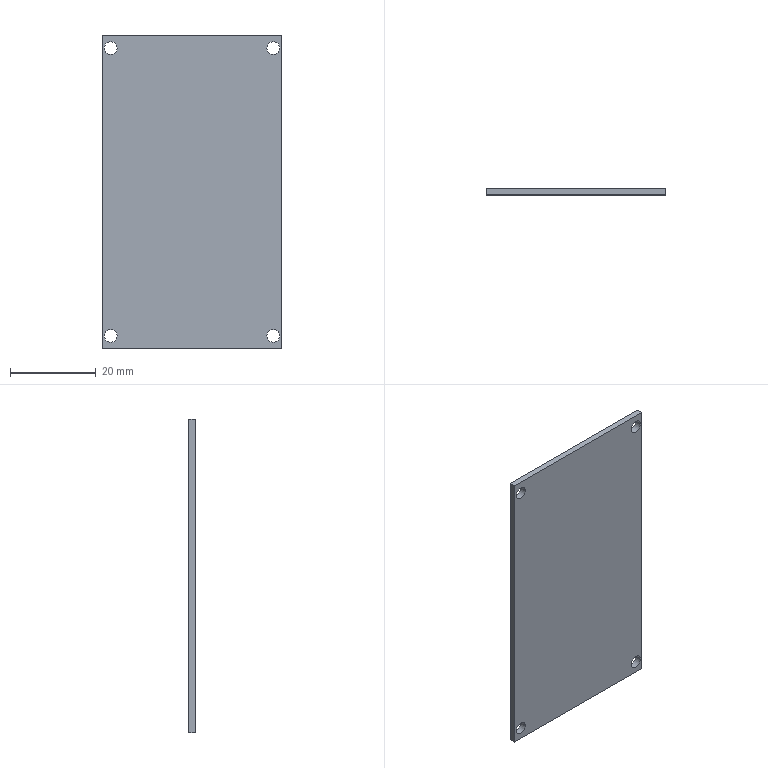Component | SolidWorks | BodyCompositionBoard-2 | 1 solid | 14 faces | box 42 x 1.5 x 73.3 mm | volume 4575 mm3 | cylinder 8 | plane 6 | commonest cylinder face diameters 3 x8
STEP:
#1=CARTESIAN_POINT('',(44.122,58.752,79.869));
#2=VERTEX_POINT('',#1);
#3=CARTESIAN_POINT('',(44.24,58.752,79.869));
#4=VERTEX_POINT('',#3);
#5=CARTESIAN_POINT('',(44.181,58.752,79.869));
#6=DIRECTION('',(0.,1.,0.));
#7=DIRECTION('',(-1.,0.,0.));
#8=AXIS2_PLACEMENT_3D('',#5,#6,#7);
#9=CIRCLE('',#8,0.05906);
#10=EDGE_CURVE('',#2,#4,#9,.T.);
#11=ORIENTED_EDGE('',*,*,#10,.F.);
#12=CARTESIAN_POINT('',(44.122,58.811,79.869));
#13=VERTEX_POINT('',#12);
#14=CARTESIAN_POINT('',(44.122,58.752,79.869));
#15=DIRECTION('',(0.,1.,0.));
#16=VECTOR('',#15,39.37);
#17=LINE('',#14,#16);
#18=EDGE_CURVE('',#2,#13,#17,.T.);
#19=ORIENTED_EDGE('',*,*,#18,.T.);
#20=CARTESIAN_POINT('',(44.24,58.811,79.869));
#21=VERTEX_POINT('',#20);
#22=CARTESIAN_POINT('',(44.181,58.811,79.869));
#23=DIRECTION('',(0.,1.,0.));
#24=DIRECTION('',(-1.,0.,0.));
#25=AXIS2_PLACEMENT_3D('',#22,#23,#24);
#26=CIRCLE('',#25,0.05906);
#27=EDGE_CURVE('',#13,#21,#26,.T.);
#28=ORIENTED_EDGE('',*,*,#27,.T.);
#29=CARTESIAN_POINT('',(44.24,58.752,79.869));
#30=DIRECTION('',(0.,1.,0.));
#31=VECTOR('',#30,39.37);
#32=LINE('',#29,#31);
#33=EDGE_CURVE('',#4,#21,#32,.T.);
#34=ORIENTED_EDGE('',*,*,#33,.F.);
#35=EDGE_LOOP('',(#11,#19,#28,#34));
#36=FACE_OUTER_BOUND('',#35,.T.);
#37=CARTESIAN_POINT('',(44.181,58.752,79.869));
#38=DIRECTION('',(0.,1.,0.));
#39=DIRECTION('',(1.,0.,0.));
#40=AXIS2_PLACEMENT_3D('',#37,#38,#39);
#41=CYLINDRICAL_SURFACE('',#40,0.05906);
#42=ADVANCED_FACE('',(#36),#41,.F.);
#43=CARTESIAN_POINT('',(45.618,58.752,79.869));
#44=VERTEX_POINT('',#43);
#45=CARTESIAN_POINT('',(45.736,58.752,79.869));
#46=VERTEX_POINT('',#45);
#47=CARTESIAN_POINT('',(45.677,58.752,79.869));
#48=DIRECTION('',(0.,1.,0.));
#49=DIRECTION('',(1.,0.,0.));
#50=AXIS2_PLACEMENT_3D('',#47,#48,#49);
#51=CIRCLE('',#50,0.05906);
#52=EDGE_CURVE('',#44,#46,#51,.T.);
#53=ORIENTED_EDGE('',*,*,#52,.F.);
#54=CARTESIAN_POINT('',(45.618,58.811,79.869));
#55=VERTEX_POINT('',#54);
#56=CARTESIAN_POINT('',(45.618,58.752,79.869));
#57=DIRECTION('',(0.,1.,0.));
#58=VECTOR('',#57,39.37);
#59=LINE('',#56,#58);
#60=EDGE_CURVE('',#44,#55,#59,.T.);
#61=ORIENTED_EDGE('',*,*,#60,.T.);
#62=CARTESIAN_POINT('',(45.736,58.811,79.869));
#63=VERTEX_POINT('',#62);
#64=CARTESIAN_POINT('',(45.677,58.811,79.869));
#65=DIRECTION('',(0.,1.,0.));
#66=DIRECTION('',(1.,0.,0.));
#67=AXIS2_PLACEMENT_3D('',#64,#65,#66);
#68=CIRCLE('',#67,0.05906);
#69=EDGE_CURVE('',#55,#63,#68,.T.);
#70=ORIENTED_EDGE('',*,*,#69,.T.);
#71=CARTESIAN_POINT('',(45.736,58.752,79.869));
#72=DIRECTION('',(0.,1.,0.));
#73=VECTOR('',#72,39.37);
#74=LINE('',#71,#73);
#75=EDGE_CURVE('',#46,#63,#74,.T.);
#76=ORIENTED_EDGE('',*,*,#75,.F.);
#77=EDGE_LOOP('',(#53,#61,#70,#76));
#78=FACE_OUTER_BOUND('',#77,.T.);
#79=CARTESIAN_POINT('',(45.677,58.752,79.869));
#80=DIRECTION('',(0.,1.,0.));
#81=DIRECTION('',(1.,0.,0.));
#82=AXIS2_PLACEMENT_3D('',#79,#80,#81);
#83=CYLINDRICAL_SURFACE('',#82,0.05906);
#84=ADVANCED_FACE('',(#78),#83,.F.);
#85=CARTESIAN_POINT('',(45.618,58.752,82.519));
#86=VERTEX_POINT('',#85);
#87=CARTESIAN_POINT('',(45.736,58.752,82.519));
#88=VERTEX_POINT('',#87);
#89=CARTESIAN_POINT('',(45.677,58.752,82.519));
#90=DIRECTION('',(0.,1.,0.));
#91=DIRECTION('',(-1.,0.,0.));
#92=AXIS2_PLACEMENT_3D('',#89,#90,#91);
#93=CIRCLE('',#92,0.05906);
#94=EDGE_CURVE('',#86,#88,#93,.T.);
#95=ORIENTED_EDGE('',*,*,#94,.F.);
#96=CARTESIAN_POINT('',(45.618,58.811,82.519));
#97=VERTEX_POINT('',#96);
#98=CARTESIAN_POINT('',(45.618,58.752,82.519));
#99=DIRECTION('',(0.,1.,0.));
#100=VECTOR('',#99,39.37);
#101=LINE('',#98,#100);
#102=EDGE_CURVE('',#86,#97,#101,.T.);
#103=ORIENTED_EDGE('',*,*,#102,.T.);
#104=CARTESIAN_POINT('',(45.736,58.811,82.519));
#105=VERTEX_POINT('',#104);
#106=CARTESIAN_POINT('',(45.677,58.811,82.519));
#107=DIRECTION('',(0.,1.,0.));
#108=DIRECTION('',(-1.,0.,0.));
#109=AXIS2_PLACEMENT_3D('',#106,#107,#108);
#110=CIRCLE('',#109,0.05906);
#111=EDGE_CURVE('',#97,#105,#110,.T.);
#112=ORIENTED_EDGE('',*,*,#111,.T.);
#113=CARTESIAN_POINT('',(45.736,58.752,82.519));
#114=DIRECTION('',(0.,1.,0.));
#115=VECTOR('',#114,39.37);
#116=LINE('',#113,#115);
#117=EDGE_CURVE('',#88,#105,#116,.T.);
#118=ORIENTED_EDGE('',*,*,#117,.F.);
#119=EDGE_LOOP('',(#95,#103,#112,#118));
#120=FACE_OUTER_BOUND('',#119,.T.);
#121=CARTESIAN_POINT('',(45.677,58.752,82.519));
#122=DIRECTION('',(0.,1.,0.));
#123=DIRECTION('',(1.,0.,0.));
#124=AXIS2_PLACEMENT_3D('',#121,#122,#123);
#125=CYLINDRICAL_SURFACE('',#124,0.05906);
#126=ADVANCED_FACE('',(#120),#125,.F.);
#127=CARTESIAN_POINT('',(44.122,58.752,82.519));
#128=VERTEX_POINT('',#127);
#129=CARTESIAN_POINT('',(44.24,58.752,82.519));
#130=VERTEX_POINT('',#129);
#131=CARTESIAN_POINT('',(44.181,58.752,82.519));
#132=DIRECTION('',(0.,1.,0.));
#133=DIRECTION('',(1.,0.,0.));
#134=AXIS2_PLACEMENT_3D('',#131,#132,#133);
#135=CIRCLE('',#134,0.05906);
#136=EDGE_CURVE('',#128,#130,#135,.T.);
#137=ORIENTED_EDGE('',*,*,#136,.F.);
#138=CARTESIAN_POINT('',(44.122,58.811,82.519));
#139=VERTEX_POINT('',#138);
#140=CARTESIAN_POINT('',(44.122,58.752,82.519));
#141=DIRECTION('',(0.,1.,0.));
#142=VECTOR('',#141,39.37);
#143=LINE('',#140,#142);
#144=EDGE_CURVE('',#128,#139,#143,.T.);
#145=ORIENTED_EDGE('',*,*,#144,.T.);
#146=CARTESIAN_POINT('',(44.24,58.811,82.519));
#147=VERTEX_POINT('',#146);
#148=CARTESIAN_POINT('',(44.181,58.811,82.519));
#149=DIRECTION('',(0.,1.,0.));
#150=DIRECTION('',(1.,0.,0.));
#151=AXIS2_PLACEMENT_3D('',#148,#149,#150);
#152=CIRCLE('',#151,0.05906);
#153=EDGE_CURVE('',#139,#147,#152,.T.);
#154=ORIENTED_EDGE('',*,*,#153,.T.);
#155=CARTESIAN_POINT('',(44.24,58.752,82.519));
#156=DIRECTION('',(0.,1.,0.));
#157=VECTOR('',#156,39.37);
#158=LINE('',#155,#157);
#159=EDGE_CURVE('',#130,#147,#158,.T.);
#160=ORIENTED_EDGE('',*,*,#159,.F.);
#161=EDGE_LOOP('',(#137,#145,#154,#160));
#162=FACE_OUTER_BOUND('',#161,.T.);
#163=CARTESIAN_POINT('',(44.181,58.752,82.519));
#164=DIRECTION('',(0.,1.,0.));
#165=DIRECTION('',(1.,0.,0.));
#166=AXIS2_PLACEMENT_3D('',#163,#164,#165);
#167=CYLINDRICAL_SURFACE('',#166,0.05906);
#168=ADVANCED_FACE('',(#162),#167,.F.);
#169=CARTESIAN_POINT('',(45.755,58.811,79.751));
#170=VERTEX_POINT('',#169);
#171=CARTESIAN_POINT('',(44.102,58.811,79.751));
#172=VERTEX_POINT('',#171);
#173=CARTESIAN_POINT('',(44.102,58.811,79.751));
#174=DIRECTION('',(-1.,0.,0.));
#175=VECTOR('',#174,39.37);
#176=LINE('',#173,#175);
#177=EDGE_CURVE('',#170,#172,#176,.T.);
#178=ORIENTED_EDGE('',*,*,#177,.F.);
#179=CARTESIAN_POINT('',(45.755,58.752,79.751));
#180=VERTEX_POINT('',#179);
#181=CARTESIAN_POINT('',(45.755,58.752,79.751));
#182=DIRECTION('',(0.,1.,0.));
#183=VECTOR('',#182,39.37);
#184=LINE('',#181,#183);
#185=EDGE_CURVE('',#180,#170,#184,.T.);
#186=ORIENTED_EDGE('',*,*,#185,.F.);
#187=CARTESIAN_POINT('',(44.102,58.752,79.751));
#188=VERTEX_POINT('',#187);
#189=CARTESIAN_POINT('',(44.102,58.752,79.751));
#190=DIRECTION('',(-1.,0.,0.));
#191=VECTOR('',#190,39.37);
#192=LINE('',#189,#191);
#193=EDGE_CURVE('',#180,#188,#192,.T.);
#194=ORIENTED_EDGE('',*,*,#193,.T.);
#195=CARTESIAN_POINT('',(44.102,58.752,79.751));
#196=DIRECTION('',(0.,1.,0.));
#197=VECTOR('',#196,39.37);
#198=LINE('',#195,#197);
#199=EDGE_CURVE('',#188,#172,#198,.T.);
#200=ORIENTED_EDGE('',*,*,#199,.T.);
#201=EDGE_LOOP('',(#178,#186,#194,#200));
#202=FACE_OUTER_BOUND('',#201,.T.);
#203=CARTESIAN_POINT('',(44.102,58.752,79.751));
#204=DIRECTION('',(-0.,0.,-1.));
#205=DIRECTION('',(-1.,0.,0.));
#206=AXIS2_PLACEMENT_3D('',#203,#204,#205);
#207=PLANE('',#206);
#208=ADVANCED_FACE('',(#202),#207,.T.);
#209=CARTESIAN_POINT('',(45.755,58.811,82.637));
#210=VERTEX_POINT('',#209);
#211=CARTESIAN_POINT('',(45.755,58.811,82.637));
#212=DIRECTION('',(-0.,0.,-1.));
#213=VECTOR('',#212,39.37);
#214=LINE('',#211,#213);
#215=EDGE_CURVE('',#210,#170,#214,.T.);
#216=ORIENTED_EDGE('',*,*,#215,.F.);
#217=CARTESIAN_POINT('',(45.755,58.752,82.637));
#218=VERTEX_POINT('',#217);
#219=CARTESIAN_POINT('',(45.755,58.752,82.637));
#220=DIRECTION('',(0.,1.,0.));
#221=VECTOR('',#220,39.37);
#222=LINE('',#219,#221);
#223=EDGE_CURVE('',#218,#210,#222,.T.);
#224=ORIENTED_EDGE('',*,*,#223,.F.);
#225=CARTESIAN_POINT('',(45.755,58.752,82.637));
#226=DIRECTION('',(-0.,0.,-1.));
#227=VECTOR('',#226,39.37);
#228=LINE('',#225,#227);
#229=EDGE_CURVE('',#218,#180,#228,.T.);
#230=ORIENTED_EDGE('',*,*,#229,.T.);
#231=ORIENTED_EDGE('',*,*,#185,.T.);
#232=EDGE_LOOP('',(#216,#224,#230,#231));
#233=FACE_OUTER_BOUND('',#232,.T.);
#234=CARTESIAN_POINT('',(45.755,58.752,82.637));
#235=DIRECTION('',(1.,0.,-0.));
#236=DIRECTION('',(-0.,0.,-1.));
#237=AXIS2_PLACEMENT_3D('',#234,#235,#236);
#238=PLANE('',#237);
#239=ADVANCED_FACE('',(#233),#238,.T.);
#240=CARTESIAN_POINT('',(44.102,58.811,82.637));
#241=VERTEX_POINT('',#240);
#242=CARTESIAN_POINT('',(44.102,58.811,82.637));
#243=DIRECTION('',(1.,0.,-0.));
#244=VECTOR('',#243,39.37);
#245=LINE('',#242,#244);
#246=EDGE_CURVE('',#241,#210,#245,.T.);
#247=ORIENTED_EDGE('',*,*,#246,.F.);
#248=CARTESIAN_POINT('',(44.102,58.752,82.637));
#249=VERTEX_POINT('',#248);
#250=CARTESIAN_POINT('',(44.102,58.752,82.637));
#251=DIRECTION('',(0.,1.,0.));
#252=VECTOR('',#251,39.37);
#253=LINE('',#250,#252);
#254=EDGE_CURVE('',#249,#241,#253,.T.);
#255=ORIENTED_EDGE('',*,*,#254,.F.);
#256=CARTESIAN_POINT('',(44.102,58.752,82.637));
#257=DIRECTION('',(1.,0.,-0.));
#258=VECTOR('',#257,39.37);
#259=LINE('',#256,#258);
#260=EDGE_CURVE('',#249,#218,#259,.T.);
#261=ORIENTED_EDGE('',*,*,#260,.T.);
#262=ORIENTED_EDGE('',*,*,#223,.T.);
#263=EDGE_LOOP('',(#247,#255,#261,#262));
#264=FACE_OUTER_BOUND('',#263,.T.);
#265=CARTESIAN_POINT('',(44.102,58.752,82.637));
#266=DIRECTION('',(0.,0.,1.));
#267=DIRECTION('',(1.,0.,-0.));
#268=AXIS2_PLACEMENT_3D('',#265,#266,#267);
#269=PLANE('',#268);
#270=ADVANCED_FACE('',(#264),#269,.T.);
#271=CARTESIAN_POINT('',(44.102,58.811,82.637));
#272=DIRECTION('',(0.,0.,1.));
#273=VECTOR('',#272,39.37);
#274=LINE('',#271,#273);
#275=EDGE_CURVE('',#172,#241,#274,.T.);
#276=ORIENTED_EDGE('',*,*,#275,.F.);
#277=ORIENTED_EDGE('',*,*,#199,.F.);
#278=CARTESIAN_POINT('',(44.102,58.752,82.637));
#279=DIRECTION('',(0.,0.,1.));
#280=VECTOR('',#279,39.37);
#281=LINE('',#278,#280);
#282=EDGE_CURVE('',#188,#249,#281,.T.);
#283=ORIENTED_EDGE('',*,*,#282,.T.);
#284=ORIENTED_EDGE('',*,*,#254,.T.);
#285=EDGE_LOOP('',(#276,#277,#283,#284));
#286=FACE_OUTER_BOUND('',#285,.T.);
#287=CARTESIAN_POINT('',(44.102,58.752,82.637));
#288=DIRECTION('',(-1.,0.,0.));
#289=DIRECTION('',(0.,0.,1.));
#290=AXIS2_PLACEMENT_3D('',#287,#288,#289);
#291=PLANE('',#290);
#292=ADVANCED_FACE('',(#286),#291,.T.);
#293=CARTESIAN_POINT('',(44.181,58.752,79.869));
#294=DIRECTION('',(0.,1.,0.));
#295=DIRECTION('',(-1.,0.,0.));
#296=AXIS2_PLACEMENT_3D('',#293,#294,#295);
#297=CIRCLE('',#296,0.05906);
#298=EDGE_CURVE('',#4,#2,#297,.T.);
#299=ORIENTED_EDGE('',*,*,#298,.T.);
#300=ORIENTED_EDGE('',*,*,#10,.T.);
#301=EDGE_LOOP('',(#299,#300));
#302=FACE_BOUND('',#301,.T.);
#303=CARTESIAN_POINT('',(45.677,58.752,79.869));
#304=DIRECTION('',(0.,1.,0.));
#305=DIRECTION('',(1.,0.,0.));
#306=AXIS2_PLACEMENT_3D('',#303,#304,#305);
#307=CIRCLE('',#306,0.05906);
#308=EDGE_CURVE('',#46,#44,#307,.T.);
#309=ORIENTED_EDGE('',*,*,#308,.T.);
#310=ORIENTED_EDGE('',*,*,#52,.T.);
#311=EDGE_LOOP('',(#309,#310));
#312=FACE_BOUND('',#311,.T.);
#313=CARTESIAN_POINT('',(45.677,58.752,82.519));
#314=DIRECTION('',(0.,1.,0.));
#315=DIRECTION('',(-1.,0.,0.));
#316=AXIS2_PLACEMENT_3D('',#313,#314,#315);
#317=CIRCLE('',#316,0.05906);
#318=EDGE_CURVE('',#88,#86,#317,.T.);
#319=ORIENTED_EDGE('',*,*,#318,.T.);
#320=ORIENTED_EDGE('',*,*,#94,.T.);
#321=EDGE_LOOP('',(#319,#320));
#322=FACE_BOUND('',#321,.T.);
#323=CARTESIAN_POINT('',(44.181,58.752,82.519));
#324=DIRECTION('',(0.,1.,0.));
#325=DIRECTION('',(1.,0.,0.));
#326=AXIS2_PLACEMENT_3D('',#323,#324,#325);
#327=CIRCLE('',#326,0.05906);
#328=EDGE_CURVE('',#130,#128,#327,.T.);
#329=ORIENTED_EDGE('',*,*,#328,.T.);
#330=ORIENTED_EDGE('',*,*,#136,.T.);
#331=EDGE_LOOP('',(#329,#330));
#332=FACE_BOUND('',#331,.T.);
#333=ORIENTED_EDGE('',*,*,#193,.F.);
#334=ORIENTED_EDGE('',*,*,#229,.F.);
#335=ORIENTED_EDGE('',*,*,#260,.F.);
#336=ORIENTED_EDGE('',*,*,#282,.F.);
#337=EDGE_LOOP('',(#333,#334,#335,#336));
#338=FACE_OUTER_BOUND('',#337,.T.);
#339=CARTESIAN_POINT('',(44.929,58.752,81.194));
#340=DIRECTION('',(0.,1.,0.));
#341=DIRECTION('',(1.,0.,-0.));
#342=AXIS2_PLACEMENT_3D('',#339,#340,#341);
#343=PLANE('',#342);
#344=ADVANCED_FACE('',(#302,#312,#322,#332,#338),#343,.F.);
#345=CARTESIAN_POINT('',(44.181,58.811,79.869));
#346=DIRECTION('',(0.,1.,0.));
#347=DIRECTION('',(-1.,0.,0.));
#348=AXIS2_PLACEMENT_3D('',#345,#346,#347);
#349=CIRCLE('',#348,0.05906);
#350=EDGE_CURVE('',#21,#13,#349,.T.);
#351=ORIENTED_EDGE('',*,*,#350,.F.);
#352=ORIENTED_EDGE('',*,*,#27,.F.);
#353=EDGE_LOOP('',(#351,#352));
#354=FACE_BOUND('',#353,.T.);
#355=CARTESIAN_POINT('',(45.677,58.811,79.869));
#356=DIRECTION('',(0.,1.,0.));
#357=DIRECTION('',(1.,0.,0.));
#358=AXIS2_PLACEMENT_3D('',#355,#356,#357);
#359=CIRCLE('',#358,0.05906);
#360=EDGE_CURVE('',#63,#55,#359,.T.);
#361=ORIENTED_EDGE('',*,*,#360,.F.);
#362=ORIENTED_EDGE('',*,*,#69,.F.);
#363=EDGE_LOOP('',(#361,#362));
#364=FACE_BOUND('',#363,.T.);
#365=CARTESIAN_POINT('',(45.677,58.811,82.519));
#366=DIRECTION('',(0.,1.,0.));
#367=DIRECTION('',(-1.,0.,0.));
#368=AXIS2_PLACEMENT_3D('',#365,#366,#367);
#369=CIRCLE('',#368,0.05906);
#370=EDGE_CURVE('',#105,#97,#369,.T.);
#371=ORIENTED_EDGE('',*,*,#370,.F.);
#372=ORIENTED_EDGE('',*,*,#111,.F.);
#373=EDGE_LOOP('',(#371,#372));
#374=FACE_BOUND('',#373,.T.);
#375=CARTESIAN_POINT('',(44.181,58.811,82.519));
#376=DIRECTION('',(0.,1.,0.));
#377=DIRECTION('',(1.,0.,0.));
#378=AXIS2_PLACEMENT_3D('',#375,#376,#377);
#379=CIRCLE('',#378,0.05906);
#380=EDGE_CURVE('',#147,#139,#379,.T.);
#381=ORIENTED_EDGE('',*,*,#380,.F.);
#382=ORIENTED_EDGE('',*,*,#153,.F.);
#383=EDGE_LOOP('',(#381,#382));
#384=FACE_BOUND('',#383,.T.);
#385=ORIENTED_EDGE('',*,*,#177,.T.);
#386=ORIENTED_EDGE('',*,*,#275,.T.);
#387=ORIENTED_EDGE('',*,*,#246,.T.);
#388=ORIENTED_EDGE('',*,*,#215,.T.);
#389=EDGE_LOOP('',(#385,#386,#387,#388));
#390=FACE_OUTER_BOUND('',#389,.T.);
#391=CARTESIAN_POINT('',(44.929,58.811,81.194));
#392=DIRECTION('',(0.,1.,0.));
#393=DIRECTION('',(1.,0.,-0.));
#394=AXIS2_PLACEMENT_3D('',#391,#392,#393);
#395=PLANE('',#394);
#396=ADVANCED_FACE('',(#354,#364,#374,#384,#390),#395,.T.);
#397=ORIENTED_EDGE('',*,*,#144,.F.);
#398=ORIENTED_EDGE('',*,*,#328,.F.);
#399=ORIENTED_EDGE('',*,*,#159,.T.);
#400=ORIENTED_EDGE('',*,*,#380,.T.);
#401=EDGE_LOOP('',(#397,#398,#399,#400));
#402=FACE_OUTER_BOUND('',#401,.T.);
#403=CARTESIAN_POINT('',(44.181,58.752,82.519));
#404=DIRECTION('',(0.,1.,0.));
#405=DIRECTION('',(1.,0.,0.));
#406=AXIS2_PLACEMENT_3D('',#403,#404,#405);
#407=CYLINDRICAL_SURFACE('',#406,0.05906);
#408=ADVANCED_FACE('',(#402),#407,.F.);
#409=ORIENTED_EDGE('',*,*,#102,.F.);
#410=ORIENTED_EDGE('',*,*,#318,.F.);
#411=ORIENTED_EDGE('',*,*,#117,.T.);
#412=ORIENTED_EDGE('',*,*,#370,.T.);
#413=EDGE_LOOP('',(#409,#410,#411,#412));
#414=FACE_OUTER_BOUND('',#413,.T.);
#415=CARTESIAN_POINT('',(45.677,58.752,82.519));
#416=DIRECTION('',(0.,1.,0.));
#417=DIRECTION('',(1.,0.,0.));
#418=AXIS2_PLACEMENT_3D('',#415,#416,#417);
#419=CYLINDRICAL_SURFACE('',#418,0.05906);
#420=ADVANCED_FACE('',(#414),#419,.F.);
#421=ORIENTED_EDGE('',*,*,#60,.F.);
#422=ORIENTED_EDGE('',*,*,#308,.F.);
#423=ORIENTED_EDGE('',*,*,#75,.T.);
#424=ORIENTED_EDGE('',*,*,#360,.T.);
#425=EDGE_LOOP('',(#421,#422,#423,#424));
#426=FACE_OUTER_BOUND('',#425,.T.);
#427=CARTESIAN_POINT('',(45.677,58.752,79.869));
#428=DIRECTION('',(0.,1.,0.));
#429=DIRECTION('',(1.,0.,0.));
#430=AXIS2_PLACEMENT_3D('',#427,#428,#429);
#431=CYLINDRICAL_SURFACE('',#430,0.05906);
#432=ADVANCED_FACE('',(#426),#431,.F.);
#433=ORIENTED_EDGE('',*,*,#18,.F.);
#434=ORIENTED_EDGE('',*,*,#298,.F.);
#435=ORIENTED_EDGE('',*,*,#33,.T.);
#436=ORIENTED_EDGE('',*,*,#350,.T.);
#437=EDGE_LOOP('',(#433,#434,#435,#436));
#438=FACE_OUTER_BOUND('',#437,.T.);
#439=CARTESIAN_POINT('',(44.181,58.752,79.869));
#440=DIRECTION('',(0.,1.,0.));
#441=DIRECTION('',(1.,0.,0.));
#442=AXIS2_PLACEMENT_3D('',#439,#440,#441);
#443=CYLINDRICAL_SURFACE('',#442,0.05906);
#444=ADVANCED_FACE('',(#438),#443,.F.);
#445=CLOSED_SHELL('',(#42,#84,#126,#168,#208,#239,#270,#292,#344,#396,#408,#420,#432,#444));
#446=MANIFOLD_SOLID_BREP('',#445);
#447=CARTESIAN_POINT('',(0.,0.,0.));
#448=DIRECTION('',(0.,0.,1.));
#449=DIRECTION('',(1.,0.,0.));
#450=AXIS2_PLACEMENT_3D('',#447,#448,#449);
#451=(LENGTH_UNIT()NAMED_UNIT(*)SI_UNIT($,.METRE.));
#452=LENGTH_MEASURE_WITH_UNIT(LENGTH_MEASURE(0.0254),#451);
#453=DIMENSIONAL_EXPONENTS(1.,0.,0.,0.,0.,0.,0.);
#454=(CONVERSION_BASED_UNIT('',#452)LENGTH_UNIT()NAMED_UNIT(#453));
#455=UNCERTAINTY_MEASURE_WITH_UNIT(LENGTH_MEASURE(0.00001),#454,'','');
#456=(NAMED_UNIT(*)PLANE_ANGLE_UNIT()SI_UNIT($,.RADIAN.));
#457=(NAMED_UNIT(*)SI_UNIT($,.STERADIAN.)SOLID_ANGLE_UNIT());
#458=(GEOMETRIC_REPRESENTATION_CONTEXT(3)GLOBAL_UNCERTAINTY_ASSIGNED_CONTEXT((#455))GLOBAL_UNIT_ASSIGNED_CONTEXT((#454,#456,#457))REPRESENTATION_CONTEXT('',''));
#459=ADVANCED_BREP_SHAPE_REPRESENTATION('',(#446,#450),#458);
#460=COLOUR_RGB('',0.7922,0.8196,0.9333);
#461=FILL_AREA_STYLE_COLOUR('',#460);
#462=FILL_AREA_STYLE('',(#461));
#463=SURFACE_STYLE_FILL_AREA(#462);
#464=SURFACE_SIDE_STYLE('',(#463));
#465=SURFACE_STYLE_USAGE(.BOTH.,#464);
#466=PRESENTATION_STYLE_ASSIGNMENT((#465));
#467=STYLED_ITEM('',(#466),#446);
#468=(LENGTH_UNIT()NAMED_UNIT(*)SI_UNIT($,.METRE.));
#469=LENGTH_MEASURE_WITH_UNIT(LENGTH_MEASURE(0.0254),#468);
#470=DIMENSIONAL_EXPONENTS(1.,0.,0.,0.,0.,0.,0.);
#471=(CONVERSION_BASED_UNIT('',#469)LENGTH_UNIT()NAMED_UNIT(#470));
#472=UNCERTAINTY_MEASURE_WITH_UNIT(LENGTH_MEASURE(0.00001),#471,'','');
#473=(NAMED_UNIT(*)PLANE_ANGLE_UNIT()SI_UNIT($,.RADIAN.));
#474=(NAMED_UNIT(*)SI_UNIT($,.STERADIAN.)SOLID_ANGLE_UNIT());
#475=(GEOMETRIC_REPRESENTATION_CONTEXT(3)GLOBAL_UNCERTAINTY_ASSIGNED_CONTEXT((#472))GLOBAL_UNIT_ASSIGNED_CONTEXT((#471,#473,#474))REPRESENTATION_CONTEXT('',''));
#476=MECHANICAL_DESIGN_GEOMETRIC_PRESENTATION_REPRESENTATION('',(#467),#475);
#477=PRESENTATION_LAYER_ASSIGNMENT('','',(#467));